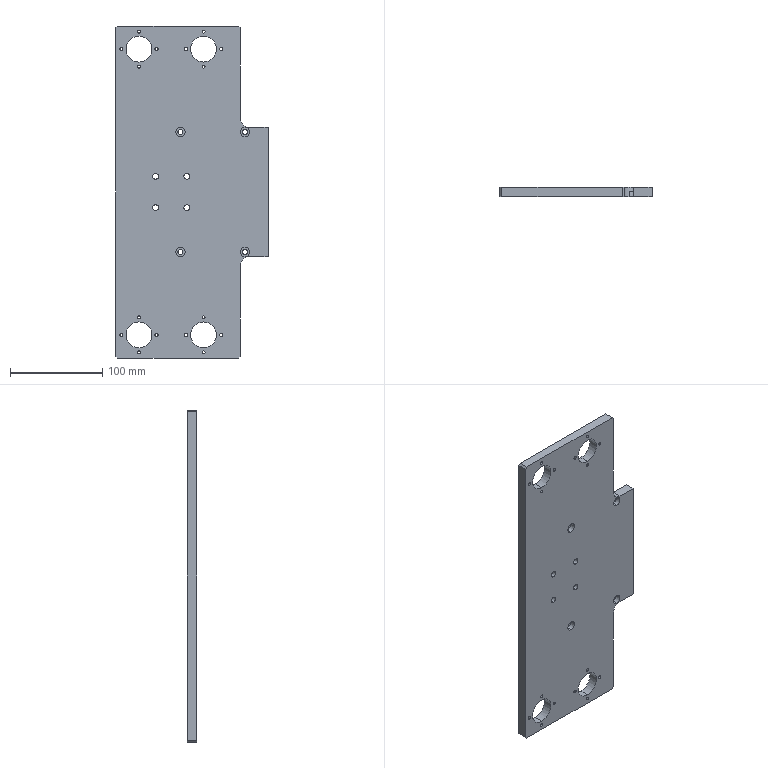Component | SolidWorks | SL021-102-4099.SL4PRT-1 | 1 solid | 100 faces | volume 497195 mm3 | cylinder 74 | plane 18 | cone 8 | commonest cylinder face diameters 3.3 x32 5 x8 6.5 x8 10 x8 5.5 x8 28.1 x8 20 x2 | material AL6061